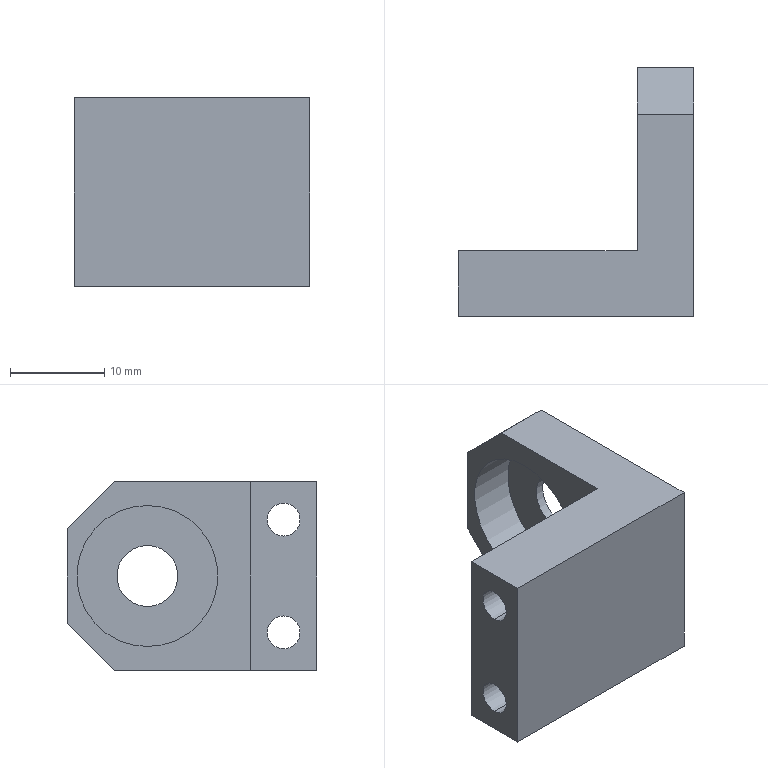Component | SolidWorks | AS-011-JG0132-1 | 1 solid | 19 faces | box 25 x 26.5 x 20 mm | volume 4292 mm3 | plane 11 | cylinder 8 | commonest cylinder face diameters 3.5 x4 15 x2 6.5 x2
build123d program:
from build123d import *

# Parameters (mm, degrees)
SKETCH1_5_W         = 20
SKETCH1_5_H         = 26.5
BOSS_EXTRUDE1_DEPTH = 6
SKETCH1_3_W         = 20
SKETCH1_3_H         = 7
SKETCH1_3_R         = 1.75
BOSS_EXTRUDE2_DEPTH = 19
CUT_EXTRUDE1_START  = 9
SKETCH1_4_R         = 1.75
CUT_EXTRUDE1_DEPTH  = 9
CUT_EXTRUDE2_START  = 5
CUT_EXTRUDE2_DEPTH  = 5
CHAMFER1_SIZE       = 5


with BuildPart() as part:
    # Sketch1_5 → Boss-Extrude1 (new body)
    with BuildSketch(Plane.XY):
        with Locations((-10, 13.25)):
            Rectangle(SKETCH1_5_W, SKETCH1_5_H)
    extrude(amount=BOSS_EXTRUDE1_DEPTH)

    # Sketch1_3 → Boss-Extrude2 (add)
    with BuildSketch(Plane.XY):
        with Locations((-10, 3.5)):
            Rectangle(SKETCH1_3_W, SKETCH1_3_H)
        with Locations((-16, 3.5)):
            Circle(SKETCH1_3_R, mode=Mode.SUBTRACT)
        with Locations((-4, 3.5)):
            Circle(SKETCH1_3_R, mode=Mode.SUBTRACT)
    extrude(amount=-BOSS_EXTRUDE2_DEPTH)

    # Sketch1_4 → Cut-Extrude1 (cut)
    with BuildSketch(Plane.XY.offset(CUT_EXTRUDE1_START)):
        with BuildLine():
            ThreePointArc((-6.75, 18), (-7.702, 20.298), (-10, 21.25))
            Line((-10, 21.25), (-10, 14.75))
            ThreePointArc((-10, 14.75), (-7.702, 15.702), (-6.75, 18))
        make_face()
        with BuildLine():
            Line((-10, 14.75), (-10, 21.25))
            ThreePointArc((-10, 21.25), (-13.25, 18), (-10, 14.75))
        make_face()
        with BuildLine():
            ThreePointArc((-6.75, 18), (-7.702, 20.298), (-10, 21.25))
            Line((-10, 21.25), (-10, 14.75))
            ThreePointArc((-10, 14.75), (-7.702, 15.702), (-6.75, 18))
        make_face()
        with BuildLine():
            Line((-10, 14.75), (-10, 21.25))
            ThreePointArc((-10, 21.25), (-13.25, 18), (-10, 14.75))
        make_face()
        with Locations((-16, 3.5)):
            Circle(SKETCH1_4_R)
        with Locations((-4, 3.5)):
            Circle(SKETCH1_4_R)
    extrude(amount=-CUT_EXTRUDE1_DEPTH, mode=Mode.SUBTRACT)

    # Sketch1_5 2 → Cut-Extrude2 (cut)
    with BuildSketch(Plane.XY.offset(CUT_EXTRUDE2_START)):
        with BuildLine():
            ThreePointArc((-2.5, 18), (-4.697, 23.303), (-10, 25.5))
            Line((-10, 25.5), (-10, 21.25))
            ThreePointArc((-10, 21.25), (-7.702, 20.298), (-6.75, 18))
            ThreePointArc((-6.75, 18), (-7.702, 15.702), (-10, 14.75))
            Line((-10, 14.75), (-10, 10.5))
            ThreePointArc((-10, 10.5), (-4.697, 12.697), (-2.5, 18))
        make_face()
        with BuildLine():
            Line((-10, 21.25), (-10, 25.5))
            ThreePointArc((-10, 25.5), (-17.5, 18), (-10, 10.5))
            Line((-10, 10.5), (-10, 14.75))
            ThreePointArc((-10, 14.75), (-13.25, 18), (-10, 21.25))
        make_face()
        with BuildLine():
            ThreePointArc((-2.5, 18), (-4.697, 23.303), (-10, 25.5))
            Line((-10, 25.5), (-10, 21.25))
            ThreePointArc((-10, 21.25), (-7.702, 20.298), (-6.75, 18))
            ThreePointArc((-6.75, 18), (-7.702, 15.702), (-10, 14.75))
            Line((-10, 14.75), (-10, 10.5))
            ThreePointArc((-10, 10.5), (-4.697, 12.697), (-2.5, 18))
        make_face()
        with BuildLine():
            Line((-10, 21.25), (-10, 25.5))
            ThreePointArc((-10, 25.5), (-17.5, 18), (-10, 10.5))
            Line((-10, 10.5), (-10, 14.75))
            ThreePointArc((-10, 14.75), (-13.25, 18), (-10, 21.25))
        make_face()
    extrude(amount=-CUT_EXTRUDE2_DEPTH, mode=Mode.SUBTRACT)

    # Chamfer1
    chamfer1_edges = [part.edges().sort_by_distance(p)[0] for p in [
        (-20, 26.5, 3),
        (0, 26.5, 3),
    ]]
    chamfer(chamfer1_edges, length=CHAMFER1_SIZE)


solid = part.part

# Placed as in the assembly
solid = solid.moved(Location((-6, -56.5, -20), (0, 90, 0)))
STEP:
#1=COLOUR_RGB('',0.7922,0.8196,0.9333);
#2=FILL_AREA_STYLE_COLOUR('',#1);
#3=FILL_AREA_STYLE('',(#2));
#4=SURFACE_STYLE_FILL_AREA(#3);
#5=SURFACE_SIDE_STYLE('',(#4));
#6=SURFACE_STYLE_USAGE(.BOTH.,#5);
#7=PRESENTATION_STYLE_ASSIGNMENT((#6));
#8=CARTESIAN_POINT('',(-0.03937,-1.516,-0.09843));
#9=VERTEX_POINT('',#8);
#10=CARTESIAN_POINT('',(-0.03937,-1.516,-0.689));
#11=VERTEX_POINT('',#10);
#12=CARTESIAN_POINT('',(-0.03937,-1.516,-0.3937));
#13=DIRECTION('',(1.,-0.,-0.));
#14=DIRECTION('',(-0.,-0.,-1.));
#15=AXIS2_PLACEMENT_3D('',#12,#13,#14);
#16=CIRCLE('',#15,0.2953);
#17=EDGE_CURVE('',#9,#11,#16,.T.);
#18=ORIENTED_EDGE('',*,*,#17,.T.);
#19=CARTESIAN_POINT('',(-0.2362,-1.516,-0.689));
#20=VERTEX_POINT('',#19);
#21=CARTESIAN_POINT('',(-0.03937,-1.516,-0.689));
#22=DIRECTION('',(-1.,0.,0.));
#23=VECTOR('',#22,39.37);
#24=LINE('',#21,#23);
#25=EDGE_CURVE('',#11,#20,#24,.T.);
#26=ORIENTED_EDGE('',*,*,#25,.T.);
#27=CARTESIAN_POINT('',(-0.2362,-1.516,-0.09843));
#28=VERTEX_POINT('',#27);
#29=CARTESIAN_POINT('',(-0.2362,-1.516,-0.3937));
#30=DIRECTION('',(1.,-0.,-0.));
#31=DIRECTION('',(0.,-0.,-1.));
#32=AXIS2_PLACEMENT_3D('',#29,#30,#31);
#33=CIRCLE('',#32,0.2953);
#34=EDGE_CURVE('',#28,#20,#33,.T.);
#35=ORIENTED_EDGE('',*,*,#34,.F.);
#36=CARTESIAN_POINT('',(-0.03937,-1.516,-0.09843));
#37=DIRECTION('',(-1.,0.,0.));
#38=VECTOR('',#37,39.37);
#39=LINE('',#36,#38);
#40=EDGE_CURVE('',#9,#28,#39,.T.);
#41=ORIENTED_EDGE('',*,*,#40,.F.);
#42=EDGE_LOOP('',(#18,#26,#35,#41));
#43=FACE_OUTER_BOUND('',#42,.T.);
#44=CARTESIAN_POINT('',(-0.03937,-1.516,-0.3937));
#45=DIRECTION('',(-1.,0.,0.));
#46=DIRECTION('',(0.,0.,1.));
#47=AXIS2_PLACEMENT_3D('',#44,#45,#46);
#48=CYLINDRICAL_SURFACE('',#47,0.2953);
#49=ADVANCED_FACE('',(#43),#48,.F.);
#50=CARTESIAN_POINT('',(-0.,-1.516,-0.5217));
#51=VERTEX_POINT('',#50);
#52=CARTESIAN_POINT('',(-0.,-1.516,-0.2657));
#53=VERTEX_POINT('',#52);
#54=CARTESIAN_POINT('',(-0.,-1.516,-0.3937));
#55=DIRECTION('',(-1.,0.,0.));
#56=DIRECTION('',(-0.,-0.,-1.));
#57=AXIS2_PLACEMENT_3D('',#54,#55,#56);
#58=CIRCLE('',#57,0.128);
#59=EDGE_CURVE('',#51,#53,#58,.T.);
#60=ORIENTED_EDGE('',*,*,#59,.F.);
#61=CARTESIAN_POINT('',(-0.03937,-1.516,-0.5217));
#62=VERTEX_POINT('',#61);
#63=CARTESIAN_POINT('',(0.1181,-1.516,-0.5217));
#64=DIRECTION('',(-1.,0.,0.));
#65=VECTOR('',#64,39.37);
#66=LINE('',#63,#65);
#67=EDGE_CURVE('',#51,#62,#66,.T.);
#68=ORIENTED_EDGE('',*,*,#67,.T.);
#69=CARTESIAN_POINT('',(-0.03937,-1.516,-0.2657));
#70=VERTEX_POINT('',#69);
#71=CARTESIAN_POINT('',(-0.03937,-1.516,-0.3937));
#72=DIRECTION('',(1.,-0.,-0.));
#73=DIRECTION('',(0.,-0.,-1.));
#74=AXIS2_PLACEMENT_3D('',#71,#72,#73);
#75=CIRCLE('',#74,0.128);
#76=EDGE_CURVE('',#70,#62,#75,.T.);
#77=ORIENTED_EDGE('',*,*,#76,.F.);
#78=CARTESIAN_POINT('',(0.1181,-1.516,-0.2657));
#79=DIRECTION('',(-1.,0.,0.));
#80=VECTOR('',#79,39.37);
#81=LINE('',#78,#80);
#82=EDGE_CURVE('',#53,#70,#81,.T.);
#83=ORIENTED_EDGE('',*,*,#82,.F.);
#84=EDGE_LOOP('',(#60,#68,#77,#83));
#85=FACE_OUTER_BOUND('',#84,.T.);
#86=CARTESIAN_POINT('',(0.1181,-1.516,-0.3937));
#87=DIRECTION('',(-1.,0.,0.));
#88=DIRECTION('',(0.,0.,1.));
#89=AXIS2_PLACEMENT_3D('',#86,#87,#88);
#90=CYLINDRICAL_SURFACE('',#89,0.128);
#91=ADVANCED_FACE('',(#85),#90,.F.);
#92=CARTESIAN_POINT('',(-0.9843,-2.087,-0.561));
#93=VERTEX_POINT('',#92);
#94=CARTESIAN_POINT('',(-0.9843,-2.087,-0.6988));
#95=VERTEX_POINT('',#94);
#96=CARTESIAN_POINT('',(-0.9843,-2.087,-0.6299));
#97=DIRECTION('',(1.,-0.,-0.));
#98=DIRECTION('',(0.,0.,-1.));
#99=AXIS2_PLACEMENT_3D('',#96,#97,#98);
#100=CIRCLE('',#99,0.0689);
#101=EDGE_CURVE('',#93,#95,#100,.T.);
#102=ORIENTED_EDGE('',*,*,#101,.F.);
#103=CARTESIAN_POINT('',(-0.,-2.087,-0.561));
#104=VERTEX_POINT('',#103);
#105=CARTESIAN_POINT('',(-0.9843,-2.087,-0.561));
#106=DIRECTION('',(1.,-0.,-0.));
#107=VECTOR('',#106,39.37);
#108=LINE('',#105,#107);
#109=EDGE_CURVE('',#93,#104,#108,.T.);
#110=ORIENTED_EDGE('',*,*,#109,.T.);
#111=CARTESIAN_POINT('',(-0.,-2.087,-0.6988));
#112=VERTEX_POINT('',#111);
#113=CARTESIAN_POINT('',(-0.,-2.087,-0.6299));
#114=DIRECTION('',(-1.,0.,0.));
#115=DIRECTION('',(-0.,-0.,-1.));
#116=AXIS2_PLACEMENT_3D('',#113,#114,#115);
#117=CIRCLE('',#116,0.0689);
#118=EDGE_CURVE('',#112,#104,#117,.T.);
#119=ORIENTED_EDGE('',*,*,#118,.F.);
#120=CARTESIAN_POINT('',(-0.9843,-2.087,-0.6988));
#121=DIRECTION('',(1.,-0.,-0.));
#122=VECTOR('',#121,39.37);
#123=LINE('',#120,#122);
#124=EDGE_CURVE('',#95,#112,#123,.T.);
#125=ORIENTED_EDGE('',*,*,#124,.F.);
#126=EDGE_LOOP('',(#102,#110,#119,#125));
#127=FACE_OUTER_BOUND('',#126,.T.);
#128=CARTESIAN_POINT('',(-0.9843,-2.087,-0.6299));
#129=DIRECTION('',(1.,-0.,-0.));
#130=DIRECTION('',(0.,0.,-1.));
#131=AXIS2_PLACEMENT_3D('',#128,#129,#130);
#132=CYLINDRICAL_SURFACE('',#131,0.0689);
#133=ADVANCED_FACE('',(#127),#132,.F.);
#134=CARTESIAN_POINT('',(-0.9843,-2.087,-0.08858));
#135=VERTEX_POINT('',#134);
#136=CARTESIAN_POINT('',(-0.9843,-2.087,-0.2264));
#137=VERTEX_POINT('',#136);
#138=CARTESIAN_POINT('',(-0.9843,-2.087,-0.1575));
#139=DIRECTION('',(1.,-0.,-0.));
#140=DIRECTION('',(0.,0.,-1.));
#141=AXIS2_PLACEMENT_3D('',#138,#139,#140);
#142=CIRCLE('',#141,0.0689);
#143=EDGE_CURVE('',#135,#137,#142,.T.);
#144=ORIENTED_EDGE('',*,*,#143,.F.);
#145=CARTESIAN_POINT('',(-0.,-2.087,-0.08858));
#146=VERTEX_POINT('',#145);
#147=CARTESIAN_POINT('',(-0.9843,-2.087,-0.08858));
#148=DIRECTION('',(1.,-0.,-0.));
#149=VECTOR('',#148,39.37);
#150=LINE('',#147,#149);
#151=EDGE_CURVE('',#135,#146,#150,.T.);
#152=ORIENTED_EDGE('',*,*,#151,.T.);
#153=CARTESIAN_POINT('',(-0.,-2.087,-0.2264));
#154=VERTEX_POINT('',#153);
#155=CARTESIAN_POINT('',(-0.,-2.087,-0.1575));
#156=DIRECTION('',(-1.,0.,0.));
#157=DIRECTION('',(-0.,-0.,-1.));
#158=AXIS2_PLACEMENT_3D('',#155,#156,#157);
#159=CIRCLE('',#158,0.0689);
#160=EDGE_CURVE('',#154,#146,#159,.T.);
#161=ORIENTED_EDGE('',*,*,#160,.F.);
#162=CARTESIAN_POINT('',(-0.9843,-2.087,-0.2264));
#163=DIRECTION('',(1.,-0.,-0.));
#164=VECTOR('',#163,39.37);
#165=LINE('',#162,#164);
#166=EDGE_CURVE('',#137,#154,#165,.T.);
#167=ORIENTED_EDGE('',*,*,#166,.F.);
#168=EDGE_LOOP('',(#144,#152,#161,#167));
#169=FACE_OUTER_BOUND('',#168,.T.);
#170=CARTESIAN_POINT('',(-0.9843,-2.087,-0.1575));
#171=DIRECTION('',(1.,-0.,-0.));
#172=DIRECTION('',(0.,0.,-1.));
#173=AXIS2_PLACEMENT_3D('',#170,#171,#172);
#174=CYLINDRICAL_SURFACE('',#173,0.0689);
#175=ADVANCED_FACE('',(#169),#174,.F.);
#176=CARTESIAN_POINT('',(-0.2362,-1.378,-0.));
#177=VERTEX_POINT('',#176);
#178=CARTESIAN_POINT('',(-0.2362,-1.949,-0.));
#179=VERTEX_POINT('',#178);
#180=CARTESIAN_POINT('',(-0.2362,-1.181,-0.));
#181=DIRECTION('',(-0.,-1.,0.));
#182=VECTOR('',#181,39.37);
#183=LINE('',#180,#182);
#184=EDGE_CURVE('',#177,#179,#183,.T.);
#185=ORIENTED_EDGE('',*,*,#184,.F.);
#186=CARTESIAN_POINT('',(-0.2362,-1.181,-0.1969));
#187=VERTEX_POINT('',#186);
#188=CARTESIAN_POINT('',(-0.2362,-1.378,-0.));
#189=DIRECTION('',(0.,0.7071,-0.7071));
#190=VECTOR('',#189,39.37);
#191=LINE('',#188,#190);
#192=EDGE_CURVE('',#177,#187,#191,.T.);
#193=ORIENTED_EDGE('',*,*,#192,.T.);
#194=CARTESIAN_POINT('',(-0.2362,-1.181,-0.5906));
#195=VERTEX_POINT('',#194);
#196=CARTESIAN_POINT('',(-0.2362,-1.181,-0.));
#197=DIRECTION('',(-0.,-0.,-1.));
#198=VECTOR('',#197,39.37);
#199=LINE('',#196,#198);
#200=EDGE_CURVE('',#187,#195,#199,.T.);
#201=ORIENTED_EDGE('',*,*,#200,.T.);
#202=CARTESIAN_POINT('',(-0.2362,-1.378,-0.7874));
#203=VERTEX_POINT('',#202);
#204=CARTESIAN_POINT('',(-0.2362,-1.181,-0.5906));
#205=DIRECTION('',(-0.,-0.7071,-0.7071));
#206=VECTOR('',#205,39.37);
#207=LINE('',#204,#206);
#208=EDGE_CURVE('',#195,#203,#207,.T.);
#209=ORIENTED_EDGE('',*,*,#208,.T.);
#210=CARTESIAN_POINT('',(-0.2362,-1.949,-0.7874));
#211=VERTEX_POINT('',#210);
#212=CARTESIAN_POINT('',(-0.2362,-1.181,-0.7874));
#213=DIRECTION('',(-0.,-1.,0.));
#214=VECTOR('',#213,39.37);
#215=LINE('',#212,#214);
#216=EDGE_CURVE('',#203,#211,#215,.T.);
#217=ORIENTED_EDGE('',*,*,#216,.T.);
#218=CARTESIAN_POINT('',(-0.2362,-1.949,-0.7874));
#219=DIRECTION('',(-0.,-0.,-1.));
#220=VECTOR('',#219,39.37);
#221=LINE('',#218,#220);
#222=EDGE_CURVE('',#179,#211,#221,.T.);
#223=ORIENTED_EDGE('',*,*,#222,.F.);
#224=EDGE_LOOP('',(#185,#193,#201,#209,#217,#223));
#225=FACE_OUTER_BOUND('',#224,.T.);
#226=ORIENTED_EDGE('',*,*,#34,.T.);
#227=CARTESIAN_POINT('',(-0.2362,-1.516,-0.3937));
#228=DIRECTION('',(1.,-0.,-0.));
#229=DIRECTION('',(0.,-0.,-1.));
#230=AXIS2_PLACEMENT_3D('',#227,#228,#229);
#231=CIRCLE('',#230,0.2953);
#232=EDGE_CURVE('',#20,#28,#231,.T.);
#233=ORIENTED_EDGE('',*,*,#232,.T.);
#234=EDGE_LOOP('',(#226,#233));
#235=FACE_BOUND('',#234,.T.);
#236=CARTESIAN_POINT('',(-0.2362,-2.224,-0.7874));
#237=DIRECTION('',(1.,-0.,-0.));
#238=DIRECTION('',(-0.,-0.,-1.));
#239=AXIS2_PLACEMENT_3D('',#236,#237,#238);
#240=PLANE('',#239);
#241=ADVANCED_FACE('',(#225,#235),#240,.F.);
#242=ORIENTED_EDGE('',*,*,#160,.T.);
#243=CARTESIAN_POINT('',(-0.,-2.087,-0.1575));
#244=DIRECTION('',(-1.,0.,0.));
#245=DIRECTION('',(-0.,-0.,-1.));
#246=AXIS2_PLACEMENT_3D('',#243,#244,#245);
#247=CIRCLE('',#246,0.0689);
#248=EDGE_CURVE('',#146,#154,#247,.T.);
#249=ORIENTED_EDGE('',*,*,#248,.T.);
#250=EDGE_LOOP('',(#242,#249));
#251=FACE_BOUND('',#250,.T.);
#252=CARTESIAN_POINT('',(-0.,-1.181,-0.1969));
#253=VERTEX_POINT('',#252);
#254=CARTESIAN_POINT('',(-0.,-1.181,-0.5906));
#255=VERTEX_POINT('',#254);
#256=CARTESIAN_POINT('',(-0.,-1.181,-0.));
#257=DIRECTION('',(-0.,-0.,-1.));
#258=VECTOR('',#257,39.37);
#259=LINE('',#256,#258);
#260=EDGE_CURVE('',#253,#255,#259,.T.);
#261=ORIENTED_EDGE('',*,*,#260,.F.);
#262=CARTESIAN_POINT('',(-0.,-1.378,-0.));
#263=VERTEX_POINT('',#262);
#264=CARTESIAN_POINT('',(-0.,-1.407,0.02953));
#265=DIRECTION('',(-0.,-0.7071,0.7071));
#266=VECTOR('',#265,39.37);
#267=LINE('',#264,#266);
#268=EDGE_CURVE('',#253,#263,#267,.T.);
#269=ORIENTED_EDGE('',*,*,#268,.T.);
#270=CARTESIAN_POINT('',(-0.,-2.224,0.));
#271=VERTEX_POINT('',#270);
#272=CARTESIAN_POINT('',(-0.,-1.181,-0.));
#273=DIRECTION('',(-0.,-1.,0.));
#274=VECTOR('',#273,39.37);
#275=LINE('',#272,#274);
#276=EDGE_CURVE('',#263,#271,#275,.T.);
#277=ORIENTED_EDGE('',*,*,#276,.T.);
#278=CARTESIAN_POINT('',(-0.,-2.224,-0.7874));
#279=VERTEX_POINT('',#278);
#280=CARTESIAN_POINT('',(-0.,-2.224,0.));
#281=DIRECTION('',(-0.,-0.,-1.));
#282=VECTOR('',#281,39.37);
#283=LINE('',#280,#282);
#284=EDGE_CURVE('',#271,#279,#283,.T.);
#285=ORIENTED_EDGE('',*,*,#284,.T.);
#286=CARTESIAN_POINT('',(-0.,-1.378,-0.7874));
#287=VERTEX_POINT('',#286);
#288=CARTESIAN_POINT('',(-0.,-1.181,-0.7874));
#289=DIRECTION('',(-0.,-1.,0.));
#290=VECTOR('',#289,39.37);
#291=LINE('',#288,#290);
#292=EDGE_CURVE('',#287,#279,#291,.T.);
#293=ORIENTED_EDGE('',*,*,#292,.F.);
#294=CARTESIAN_POINT('',(-0.,-1.801,-1.211));
#295=DIRECTION('',(0.,0.7071,0.7071));
#296=VECTOR('',#295,39.37);
#297=LINE('',#294,#296);
#298=EDGE_CURVE('',#287,#255,#297,.T.);
#299=ORIENTED_EDGE('',*,*,#298,.T.);
#300=EDGE_LOOP('',(#261,#269,#277,#285,#293,#299));
#301=FACE_OUTER_BOUND('',#300,.T.);
#302=CARTESIAN_POINT('',(-0.,-1.516,-0.3937));
#303=DIRECTION('',(-1.,0.,0.));
#304=DIRECTION('',(-0.,-0.,-1.));
#305=AXIS2_PLACEMENT_3D('',#302,#303,#304);
#306=CIRCLE('',#305,0.128);
#307=EDGE_CURVE('',#53,#51,#306,.T.);
#308=ORIENTED_EDGE('',*,*,#307,.T.);
#309=ORIENTED_EDGE('',*,*,#59,.T.);
#310=EDGE_LOOP('',(#308,#309));
#311=FACE_BOUND('',#310,.T.);
#312=ORIENTED_EDGE('',*,*,#118,.T.);
#313=CARTESIAN_POINT('',(-0.,-2.087,-0.6299));
#314=DIRECTION('',(-1.,0.,0.));
#315=DIRECTION('',(-0.,-0.,-1.));
#316=AXIS2_PLACEMENT_3D('',#313,#314,#315);
#317=CIRCLE('',#316,0.0689);
#318=EDGE_CURVE('',#104,#112,#317,.T.);
#319=ORIENTED_EDGE('',*,*,#318,.T.);
#320=EDGE_LOOP('',(#312,#319));
#321=FACE_BOUND('',#320,.T.);
#322=CARTESIAN_POINT('',(-0.,-2.224,-0.7874));
#323=DIRECTION('',(1.,-0.,-0.));
#324=DIRECTION('',(-0.,-0.,-1.));
#325=AXIS2_PLACEMENT_3D('',#322,#323,#324);
#326=PLANE('',#325);
#327=ADVANCED_FACE('',(#251,#301,#311,#321),#326,.T.);
#328=ORIENTED_EDGE('',*,*,#276,.F.);
#329=CARTESIAN_POINT('',(-0.2362,-1.378,-0.));
#330=DIRECTION('',(-1.,0.,0.));
#331=VECTOR('',#330,39.37);
#332=LINE('',#329,#331);
#333=EDGE_CURVE('',#263,#177,#332,.T.);
#334=ORIENTED_EDGE('',*,*,#333,.T.);
#335=ORIENTED_EDGE('',*,*,#184,.T.);
#336=CARTESIAN_POINT('',(-0.9843,-1.949,-0.));
#337=VERTEX_POINT('',#336);
#338=CARTESIAN_POINT('',(-0.9843,-1.949,-0.));
#339=DIRECTION('',(1.,-0.,-0.));
#340=VECTOR('',#339,39.37);
#341=LINE('',#338,#340);
#342=EDGE_CURVE('',#337,#179,#341,.T.);
#343=ORIENTED_EDGE('',*,*,#342,.F.);
#344=CARTESIAN_POINT('',(-0.9843,-2.224,0.));
#345=VERTEX_POINT('',#344);
#346=CARTESIAN_POINT('',(-0.9843,-2.224,0.));
#347=DIRECTION('',(-0.,-1.,0.));
#348=VECTOR('',#347,39.37);
#349=LINE('',#346,#348);
#350=EDGE_CURVE('',#337,#345,#349,.T.);
#351=ORIENTED_EDGE('',*,*,#350,.T.);
#352=CARTESIAN_POINT('',(-0.,-2.224,0.));
#353=DIRECTION('',(-1.,0.,0.));
#354=VECTOR('',#353,39.37);
#355=LINE('',#352,#354);
#356=EDGE_CURVE('',#271,#345,#355,.T.);
#357=ORIENTED_EDGE('',*,*,#356,.F.);
#358=EDGE_LOOP('',(#328,#334,#335,#343,#351,#357));
#359=FACE_OUTER_BOUND('',#358,.T.);
#360=CARTESIAN_POINT('',(-0.,-1.181,-0.));
#361=DIRECTION('',(-0.,-0.,-1.));
#362=DIRECTION('',(-1.,0.,0.));
#363=AXIS2_PLACEMENT_3D('',#360,#361,#362);
#364=PLANE('',#363);
#365=ADVANCED_FACE('',(#359),#364,.F.);
#366=ORIENTED_EDGE('',*,*,#356,.T.);
#367=CARTESIAN_POINT('',(-0.9843,-2.224,-0.7874));
#368=VERTEX_POINT('',#367);
#369=CARTESIAN_POINT('',(-0.9843,-2.224,-0.7874));
#370=DIRECTION('',(-0.,-0.,-1.));
#371=VECTOR('',#370,39.37);
#372=LINE('',#369,#371);
#373=EDGE_CURVE('',#345,#368,#372,.T.);
#374=ORIENTED_EDGE('',*,*,#373,.T.);
#375=CARTESIAN_POINT('',(-0.,-2.224,-0.7874));
#376=DIRECTION('',(-1.,0.,0.));
#377=VECTOR('',#376,39.37);
#378=LINE('',#375,#377);
#379=EDGE_CURVE('',#279,#368,#378,.T.);
#380=ORIENTED_EDGE('',*,*,#379,.F.);
#381=ORIENTED_EDGE('',*,*,#284,.F.);
#382=EDGE_LOOP('',(#366,#374,#380,#381));
#383=FACE_OUTER_BOUND('',#382,.T.);
#384=CARTESIAN_POINT('',(-0.,-2.224,0.));
#385=DIRECTION('',(0.,1.,-0.));
#386=DIRECTION('',(1.,-0.,-0.));
#387=AXIS2_PLACEMENT_3D('',#384,#385,#386);
#388=PLANE('',#387);
#389=ADVANCED_FACE('',(#383),#388,.F.);
#390=ORIENTED_EDGE('',*,*,#216,.F.);
#391=CARTESIAN_POINT('',(-0.,-1.378,-0.7874));
#392=DIRECTION('',(1.,-0.,-0.));
#393=VECTOR('',#392,39.37);
#394=LINE('',#391,#393);
#395=EDGE_CURVE('',#203,#287,#394,.T.);
#396=ORIENTED_EDGE('',*,*,#395,.T.);
#397=ORIENTED_EDGE('',*,*,#292,.T.);
#398=ORIENTED_EDGE('',*,*,#379,.T.);
#399=CARTESIAN_POINT('',(-0.9843,-1.949,-0.7874));
#400=VERTEX_POINT('',#399);
#401=CARTESIAN_POINT('',(-0.9843,-2.224,-0.7874));
#402=DIRECTION('',(-0.,-1.,0.));
#403=VECTOR('',#402,39.37);
#404=LINE('',#401,#403);
#405=EDGE_CURVE('',#400,#368,#404,.T.);
#406=ORIENTED_EDGE('',*,*,#405,.F.);
#407=CARTESIAN_POINT('',(-0.9843,-1.949,-0.7874));
#408=DIRECTION('',(1.,-0.,-0.));
#409=VECTOR('',#408,39.37);
#410=LINE('',#407,#409);
#411=EDGE_CURVE('',#400,#211,#410,.T.);
#412=ORIENTED_EDGE('',*,*,#411,.T.);
#413=EDGE_LOOP('',(#390,#396,#397,#398,#406,#412));
#414=FACE_OUTER_BOUND('',#413,.T.);
#415=CARTESIAN_POINT('',(-0.,-1.181,-0.7874));
#416=DIRECTION('',(-0.,-0.,-1.));
#417=DIRECTION('',(-1.,0.,0.));
#418=AXIS2_PLACEMENT_3D('',#415,#416,#417);
#419=PLANE('',#418);
#420=ADVANCED_FACE('',(#414),#419,.T.);
#421=ORIENTED_EDGE('',*,*,#200,.F.);
#422=CARTESIAN_POINT('',(-0.,-1.181,-0.1969));
#423=DIRECTION('',(1.,-0.,-0.));
#424=VECTOR('',#423,39.37);
#425=LINE('',#422,#424);
#426=EDGE_CURVE('',#187,#253,#425,.T.);
#427=ORIENTED_EDGE('',*,*,#426,.T.);
#428=ORIENTED_EDGE('',*,*,#260,.T.);
#429=CARTESIAN_POINT('',(-0.,-1.181,-0.5906));
#430=DIRECTION('',(-1.,0.,0.));
#431=VECTOR('',#430,39.37);
#432=LINE('',#429,#431);
#433=EDGE_CURVE('',#255,#195,#432,.T.);
#434=ORIENTED_EDGE('',*,*,#433,.T.);
#435=EDGE_LOOP('',(#421,#427,#428,#434));
#436=FACE_OUTER_BOUND('',#435,.T.);
#437=CARTESIAN_POINT('',(-0.,-1.181,-0.));
#438=DIRECTION('',(0.,1.,-0.));
#439=DIRECTION('',(1.,-0.,-0.));
#440=AXIS2_PLACEMENT_3D('',#437,#438,#439);
#441=PLANE('',#440);
#442=ADVANCED_FACE('',(#436),#441,.T.);
#443=ORIENTED_EDGE('',*,*,#222,.T.);
#444=ORIENTED_EDGE('',*,*,#411,.F.);
#445=CARTESIAN_POINT('',(-0.9843,-1.949,-0.7874));
#446=DIRECTION('',(-0.,-0.,-1.));
#447=VECTOR('',#446,39.37);
#448=LINE('',#445,#447);
#449=EDGE_CURVE('',#337,#400,#448,.T.);
#450=ORIENTED_EDGE('',*,*,#449,.F.);
#451=ORIENTED_EDGE('',*,*,#342,.T.);
#452=EDGE_LOOP('',(#443,#444,#450,#451));
#453=FACE_OUTER_BOUND('',#452,.T.);
#454=CARTESIAN_POINT('',(-0.9843,-1.949,-0.7874));
#455=DIRECTION('',(-0.,-1.,0.));
#456=DIRECTION('',(-1.,0.,0.));
#457=AXIS2_PLACEMENT_3D('',#454,#455,#456);
#458=PLANE('',#457);
#459=ADVANCED_FACE('',(#453),#458,.F.);
#460=ORIENTED_EDGE('',*,*,#151,.F.);
#461=CARTESIAN_POINT('',(-0.9843,-2.087,-0.1575));
#462=DIRECTION('',(1.,-0.,-0.));
#463=DIRECTION('',(0.,0.,-1.));
#464=AXIS2_PLACEMENT_3D('',#461,#462,#463);
#465=CIRCLE('',#464,0.0689);
#466=EDGE_CURVE('',#137,#135,#465,.T.);
#467=ORIENTED_EDGE('',*,*,#466,.F.);
#468=ORIENTED_EDGE('',*,*,#166,.T.);
#469=ORIENTED_EDGE('',*,*,#248,.F.);
#470=EDGE_LOOP('',(#460,#467,#468,#469));
#471=FACE_OUTER_BOUND('',#470,.T.);
#472=CARTESIAN_POINT('',(-0.9843,-2.087,-0.1575));
#473=DIRECTION('',(1.,-0.,-0.));
#474=DIRECTION('',(0.,0.,-1.));
#475=AXIS2_PLACEMENT_3D('',#472,#473,#474);
#476=CYLINDRICAL_SURFACE('',#475,0.0689);
#477=ADVANCED_FACE('',(#471),#476,.F.);
#478=ORIENTED_EDGE('',*,*,#109,.F.);
#479=CARTESIAN_POINT('',(-0.9843,-2.087,-0.6299));
#480=DIRECTION('',(1.,-0.,-0.));
#481=DIRECTION('',(0.,0.,-1.));
#482=AXIS2_PLACEMENT_3D('',#479,#480,#481);
#483=CIRCLE('',#482,0.0689);
#484=EDGE_CURVE('',#95,#93,#483,.T.);
#485=ORIENTED_EDGE('',*,*,#484,.F.);
#486=ORIENTED_EDGE('',*,*,#124,.T.);
#487=ORIENTED_EDGE('',*,*,#318,.F.);
#488=EDGE_LOOP('',(#478,#485,#486,#487));
#489=FACE_OUTER_BOUND('',#488,.T.);
#490=CARTESIAN_POINT('',(-0.9843,-2.087,-0.6299));
#491=DIRECTION('',(1.,-0.,-0.));
#492=DIRECTION('',(0.,0.,-1.));
#493=AXIS2_PLACEMENT_3D('',#490,#491,#492);
#494=CYLINDRICAL_SURFACE('',#493,0.0689);
#495=ADVANCED_FACE('',(#489),#494,.F.);
#496=ORIENTED_EDGE('',*,*,#484,.T.);
#497=ORIENTED_EDGE('',*,*,#101,.T.);
#498=EDGE_LOOP('',(#496,#497));
#499=FACE_BOUND('',#498,.T.);
#500=ORIENTED_EDGE('',*,*,#466,.T.);
#501=ORIENTED_EDGE('',*,*,#143,.T.);
#502=EDGE_LOOP('',(#500,#501));
#503=FACE_BOUND('',#502,.T.);
#504=ORIENTED_EDGE('',*,*,#449,.T.);
#505=ORIENTED_EDGE('',*,*,#405,.T.);
#506=ORIENTED_EDGE('',*,*,#373,.F.);
#507=ORIENTED_EDGE('',*,*,#350,.F.);
#508=EDGE_LOOP('',(#504,#505,#506,#507));
#509=FACE_OUTER_BOUND('',#508,.T.);
#510=CARTESIAN_POINT('',(-0.9843,-2.224,-0.7874));
#511=DIRECTION('',(1.,-0.,-0.));
#512=DIRECTION('',(-0.,-0.,-1.));
#513=AXIS2_PLACEMENT_3D('',#510,#511,#512);
#514=PLANE('',#513);
#515=ADVANCED_FACE('',(#499,#503,#509),#514,.F.);
#516=ORIENTED_EDGE('',*,*,#67,.F.);
#517=ORIENTED_EDGE('',*,*,#307,.F.);
#518=ORIENTED_EDGE('',*,*,#82,.T.);
#519=CARTESIAN_POINT('',(-0.03937,-1.516,-0.3937));
#520=DIRECTION('',(1.,-0.,-0.));
#521=DIRECTION('',(0.,-0.,-1.));
#522=AXIS2_PLACEMENT_3D('',#519,#520,#521);
#523=CIRCLE('',#522,0.128);
#524=EDGE_CURVE('',#62,#70,#523,.T.);
#525=ORIENTED_EDGE('',*,*,#524,.F.);
#526=EDGE_LOOP('',(#516,#517,#518,#525));
#527=FACE_OUTER_BOUND('',#526,.T.);
#528=CARTESIAN_POINT('',(0.1181,-1.516,-0.3937));
#529=DIRECTION('',(-1.,0.,0.));
#530=DIRECTION('',(0.,0.,1.));
#531=AXIS2_PLACEMENT_3D('',#528,#529,#530);
#532=CYLINDRICAL_SURFACE('',#531,0.128);
#533=ADVANCED_FACE('',(#527),#532,.F.);
#534=ORIENTED_EDGE('',*,*,#25,.F.);
#535=CARTESIAN_POINT('',(-0.03937,-1.516,-0.3937));
#536=DIRECTION('',(1.,-0.,-0.));
#537=DIRECTION('',(-0.,-0.,-1.));
#538=AXIS2_PLACEMENT_3D('',#535,#536,#537);
#539=CIRCLE('',#538,0.2953);
#540=EDGE_CURVE('',#11,#9,#539,.T.);
#541=ORIENTED_EDGE('',*,*,#540,.T.);
#542=ORIENTED_EDGE('',*,*,#40,.T.);
#543=ORIENTED_EDGE('',*,*,#232,.F.);
#544=EDGE_LOOP('',(#534,#541,#542,#543));
#545=FACE_OUTER_BOUND('',#544,.T.);
#546=CARTESIAN_POINT('',(-0.03937,-1.516,-0.3937));
#547=DIRECTION('',(-1.,0.,0.));
#548=DIRECTION('',(0.,0.,1.));
#549=AXIS2_PLACEMENT_3D('',#546,#547,#548);
#550=CYLINDRICAL_SURFACE('',#549,0.2953);
#551=ADVANCED_FACE('',(#545),#550,.F.);
#552=ORIENTED_EDGE('',*,*,#76,.T.);
#553=ORIENTED_EDGE('',*,*,#524,.T.);
#554=EDGE_LOOP('',(#552,#553));
#555=FACE_BOUND('',#554,.T.);
#556=ORIENTED_EDGE('',*,*,#17,.F.);
#557=ORIENTED_EDGE('',*,*,#540,.F.);
#558=EDGE_LOOP('',(#556,#557));
#559=FACE_OUTER_BOUND('',#558,.T.);
#560=CARTESIAN_POINT('',(-0.03937,-2.224,-0.7874));
#561=DIRECTION('',(1.,-0.,-0.));
#562=DIRECTION('',(-0.,-0.,-1.));
#563=AXIS2_PLACEMENT_3D('',#560,#561,#562);
#564=PLANE('',#563);
#565=ADVANCED_FACE('',(#555,#559),#564,.F.);
#566=ORIENTED_EDGE('',*,*,#268,.F.);
#567=ORIENTED_EDGE('',*,*,#426,.F.);
#568=ORIENTED_EDGE('',*,*,#192,.F.);
#569=ORIENTED_EDGE('',*,*,#333,.F.);
#570=EDGE_LOOP('',(#566,#567,#568,#569));
#571=FACE_OUTER_BOUND('',#570,.T.);
#572=CARTESIAN_POINT('',(-0.,-1.378,-0.));
#573=DIRECTION('',(0.,0.7071,0.7071));
#574=DIRECTION('',(1.,-0.,-0.));
#575=AXIS2_PLACEMENT_3D('',#572,#573,#574);
#576=PLANE('',#575);
#577=ADVANCED_FACE('',(#571),#576,.T.);
#578=ORIENTED_EDGE('',*,*,#298,.F.);
#579=ORIENTED_EDGE('',*,*,#395,.F.);
#580=ORIENTED_EDGE('',*,*,#208,.F.);
#581=ORIENTED_EDGE('',*,*,#433,.F.);
#582=EDGE_LOOP('',(#578,#579,#580,#581));
#583=FACE_OUTER_BOUND('',#582,.T.);
#584=CARTESIAN_POINT('',(-0.,-1.181,-0.5906));
#585=DIRECTION('',(-0.,-0.7071,0.7071));
#586=DIRECTION('',(-1.,0.,0.));
#587=AXIS2_PLACEMENT_3D('',#584,#585,#586);
#588=PLANE('',#587);
#589=ADVANCED_FACE('',(#583),#588,.F.);
#590=CLOSED_SHELL('',(#49,#91,#133,#175,#241,#327,#365,#389,#420,#442,#459,#477,#495,#515,#533,#551,#565,#577,#589));
#591=MANIFOLD_SOLID_BREP('',#590);
#592=STYLED_ITEM('',(#7),#591);
#593=PRESENTATION_LAYER_ASSIGNMENT('','',(#592));
#594=(LENGTH_UNIT()NAMED_UNIT(*)SI_UNIT($,.METRE.));
#595=LENGTH_MEASURE_WITH_UNIT(LENGTH_MEASURE(0.0254),#594);
#596=DIMENSIONAL_EXPONENTS(1.,0.,0.,0.,0.,0.,0.);
#597=(CONVERSION_BASED_UNIT('',#595)LENGTH_UNIT()NAMED_UNIT(#596));
#598=UNCERTAINTY_MEASURE_WITH_UNIT(LENGTH_MEASURE(0.00001),#597,'','');
#599=(NAMED_UNIT(*)PLANE_ANGLE_UNIT()SI_UNIT($,.RADIAN.));
#600=(NAMED_UNIT(*)SI_UNIT($,.STERADIAN.)SOLID_ANGLE_UNIT());
#601=(GEOMETRIC_REPRESENTATION_CONTEXT(3)GLOBAL_UNCERTAINTY_ASSIGNED_CONTEXT((#598))GLOBAL_UNIT_ASSIGNED_CONTEXT((#597,#599,#600))REPRESENTATION_CONTEXT('',''));
#602=MECHANICAL_DESIGN_GEOMETRIC_PRESENTATION_REPRESENTATION('',(#592),#601);
#603=CARTESIAN_POINT('',(0.,0.,0.));
#604=DIRECTION('',(0.,0.,1.));
#605=DIRECTION('',(1.,0.,0.));
#606=AXIS2_PLACEMENT_3D('',#603,#604,#605);
#607=(LENGTH_UNIT()NAMED_UNIT(*)SI_UNIT($,.METRE.));
#608=LENGTH_MEASURE_WITH_UNIT(LENGTH_MEASURE(0.0254),#607);
#609=DIMENSIONAL_EXPONENTS(1.,0.,0.,0.,0.,0.,0.);
#610=(CONVERSION_BASED_UNIT('',#608)LENGTH_UNIT()NAMED_UNIT(#609));
#611=UNCERTAINTY_MEASURE_WITH_UNIT(LENGTH_MEASURE(0.00001),#610,'','');
#612=(NAMED_UNIT(*)PLANE_ANGLE_UNIT()SI_UNIT($,.RADIAN.));
#613=(NAMED_UNIT(*)SI_UNIT($,.STERADIAN.)SOLID_ANGLE_UNIT());
#614=(GEOMETRIC_REPRESENTATION_CONTEXT(3)GLOBAL_UNCERTAINTY_ASSIGNED_CONTEXT((#611))GLOBAL_UNIT_ASSIGNED_CONTEXT((#610,#612,#613))REPRESENTATION_CONTEXT('',''));
#615=ADVANCED_BREP_SHAPE_REPRESENTATION('',(#591,#606),#614);